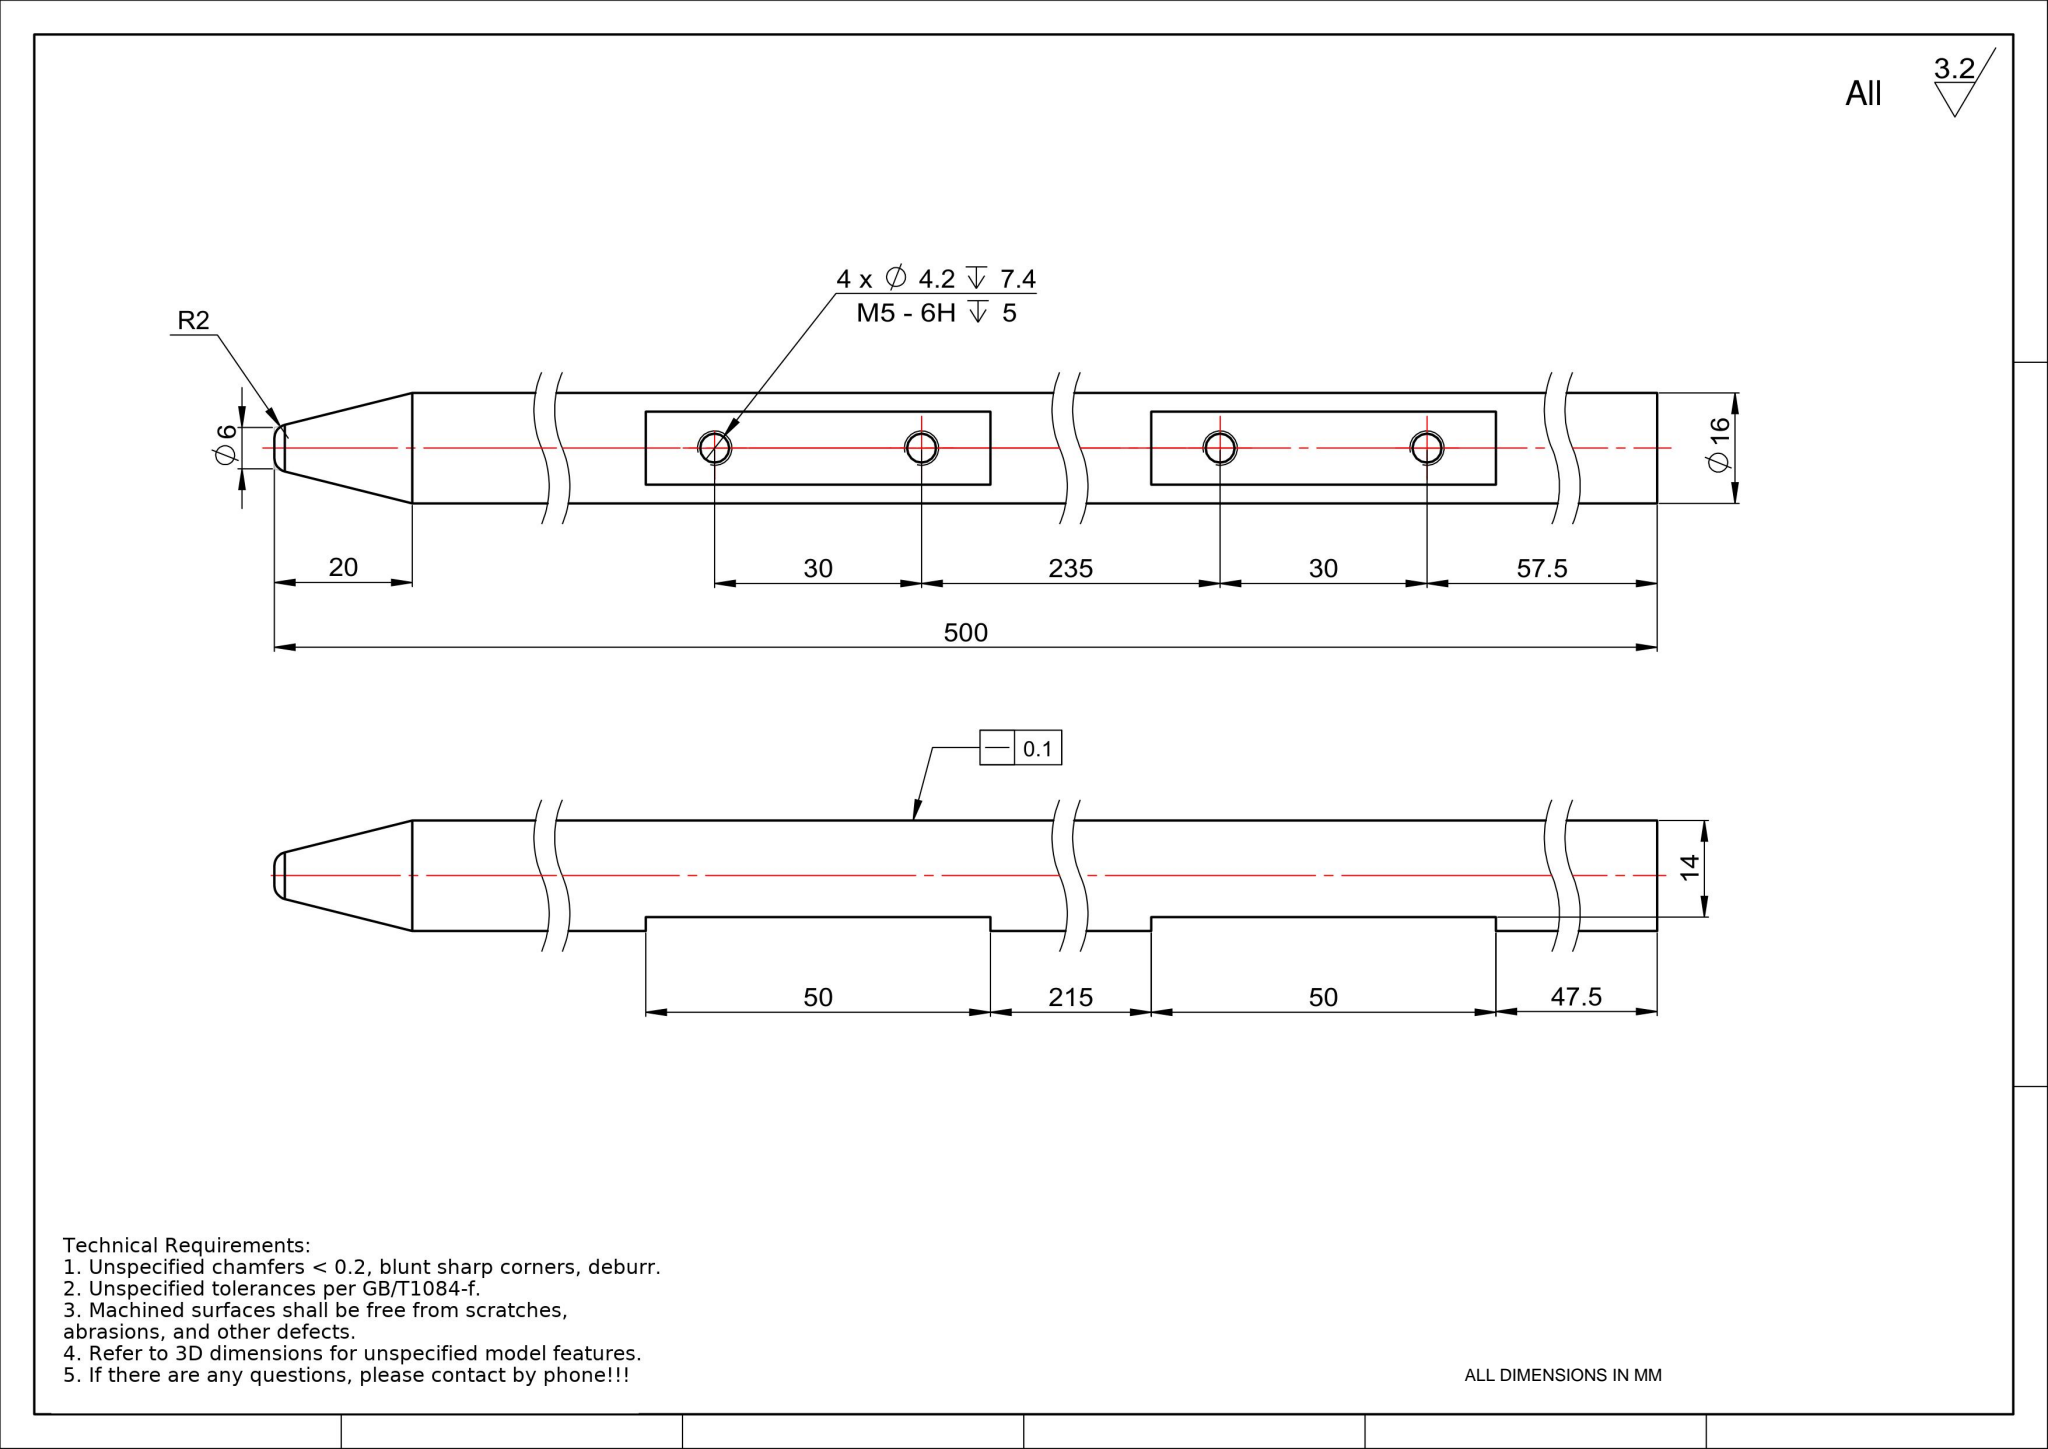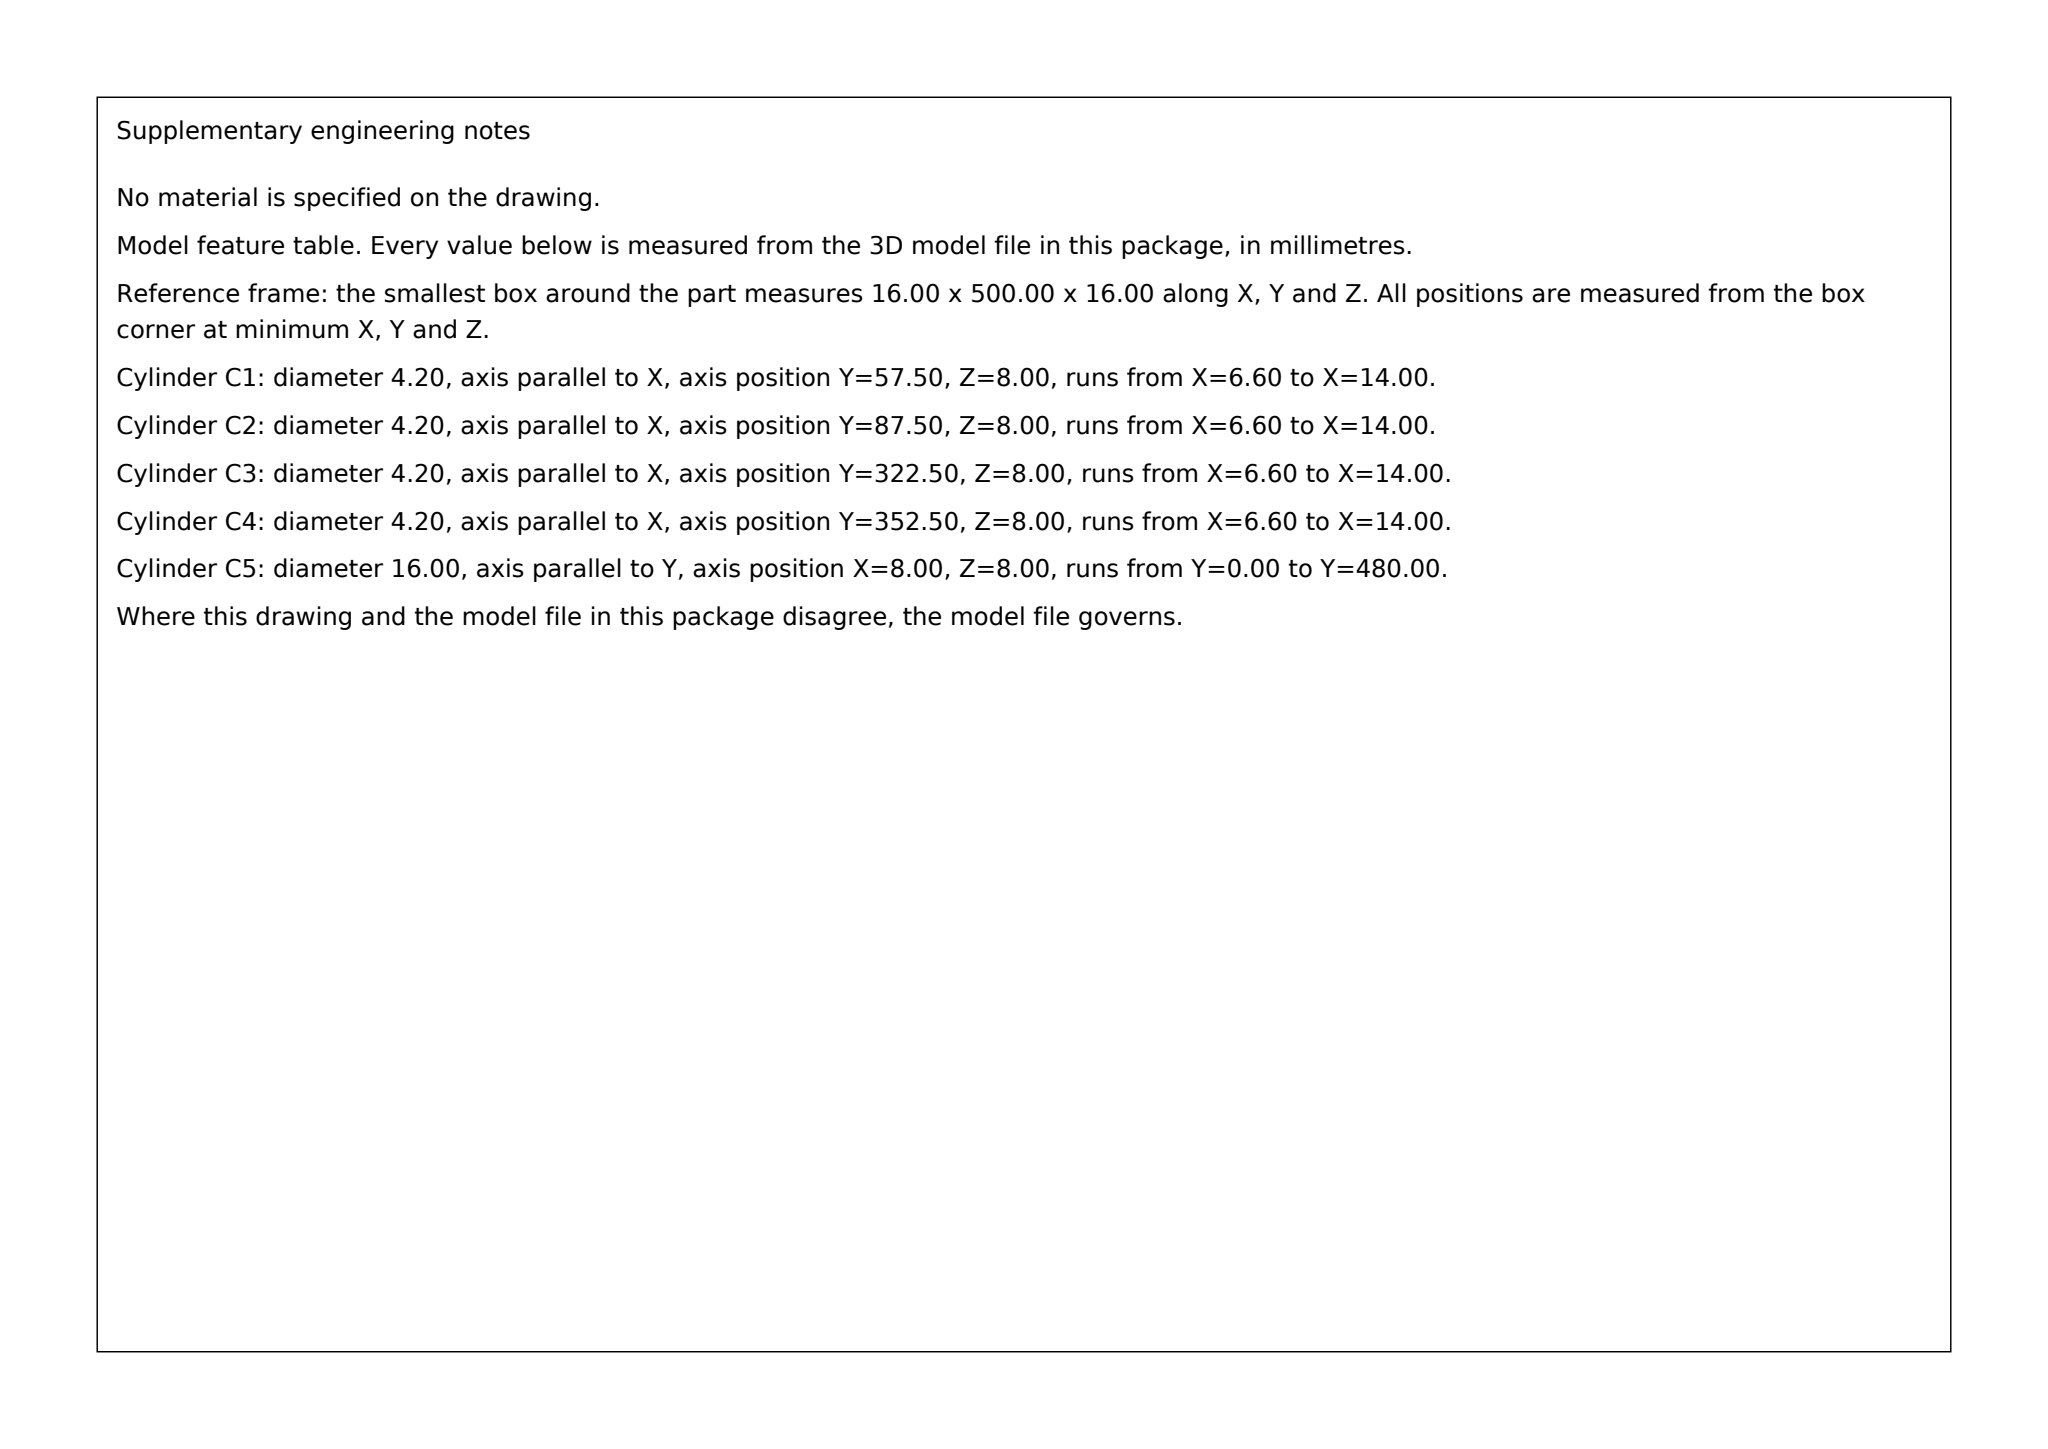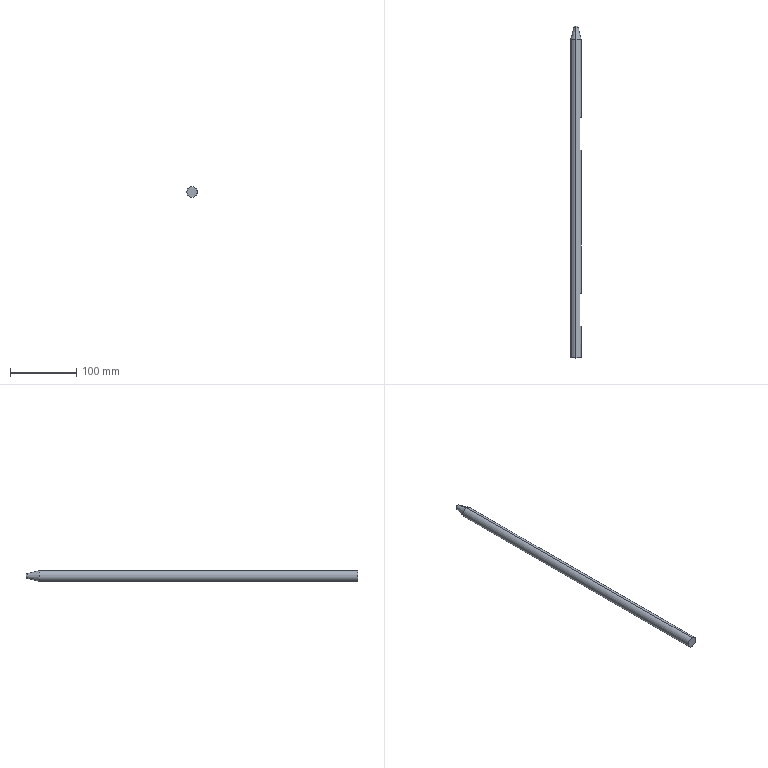Part | SolidWorks | mm | 1 solid | 30 faces | box 16 x 500 x 16 mm | volume 96649 mm3 | cylinder 10 | cone 10 | plane 8 | torus 2 | commonest cylinder face diameters 4.2 x8 16 x2
build123d program:
from build123d import *

# Parameters (mm, degrees)
SKETCH1_R                  = 8
BOSS_EXTRUDE1_DEPTH        = 500
CHAMFER2_SIZE              = 20
CHAMFER2_SIZE2             = 5
CUT_EXTRUDE1_START         = 6
SKETCH2_W                  = 36.807
SKETCH2_H                  = 50
CUT_EXTRUDE1_DEPTH         = 11
M5_TAPPED_HOLE1_AT_2_COUNT = 2
M5_TAPPED_HOLE1_AT_2_PITCH = 30
FILLET1_R                  = 2
LPATTERN3_COUNT            = 2
LPATTERN3_PITCH            = 265


with BuildPart() as part:
    # Sketch1 → Boss-Extrude1 (new body)
    with BuildSketch(Plane(origin=(0, 0, 0), x_dir=(1, 0, 0), z_dir=(0, 1, 0))):
        with Locations(Location((0, 0, 0), (0, 0, 270))):
            Circle(SKETCH1_R)
    extrude(amount=BOSS_EXTRUDE1_DEPTH)

    # Chamfer2
    chamfer2_edges = [part.edges().sort_by_distance(p)[0] for p in [
        (0, 500, -8),
    ]]
    chamfer2_side = [part.faces().sort_by_distance(p)[0] for p in [
        (0, 250, -8),
    ]]
    chamfer(chamfer2_edges, length=CHAMFER2_SIZE, length2=CHAMFER2_SIZE2, reference=chamfer2_side[0])

    # Sketch2 → Cut-Extrude1 (cut)
    with BuildSketch(Plane(origin=(0, 0, 0), x_dir=(0, 0, -1), z_dir=(1, 0, 0)).offset(CUT_EXTRUDE1_START)):
        with Locations((0, 72.5)):
            Rectangle(SKETCH2_W, SKETCH2_H)
    cut_extrude1 = extrude(amount=CUT_EXTRUDE1_DEPTH, mode=Mode.SUBTRACT)

    # Sketch3 → M5 Tapped Hole1 (revolve, cut)
    with BuildSketch(Plane(origin=(6, 87.5, 0), x_dir=(0, 0, -1), z_dir=(0, 1, 0))):
        Polygon((0, 0), (0, 8.662), (2.1, 7.4), (2.1, 0), align=None)
    m5_tapped_hole1 = revolve(axis=Axis((12.35, 87.5, 0), (-1, 0, 0)), mode=Mode.SUBTRACT)

    # M5 Tapped Hole1 at 2: M5 Tapped Hole1 ×2
    with Locations(*[(0, -i * M5_TAPPED_HOLE1_AT_2_PITCH, 0) for i in range(1, M5_TAPPED_HOLE1_AT_2_COUNT)]):
        add(m5_tapped_hole1, mode=Mode.SUBTRACT)

    # Fillet1
    fillet1_edges = [part.edges().sort_by_distance(p)[0] for p in [
        (0, 500, -3),
    ]]
    fillet(fillet1_edges, radius=FILLET1_R)

    # LPattern3: Cut-Extrude1, M5 Tapped Hole1 ×2
    with Locations(*[(0, i * LPATTERN3_PITCH, 0) for i in range(1, LPATTERN3_COUNT)]):
        add(cut_extrude1, mode=Mode.SUBTRACT)
        add(m5_tapped_hole1, mode=Mode.SUBTRACT)

    # LPattern3 copy 1 sketch → LPattern3 copy 1 (revolve, cut)
    with BuildSketch(Plane(origin=(6, 322.5, 0), x_dir=(0, 0, -1), z_dir=(0, 1, 0))):
        Polygon((0, 0), (0, 8.662), (2.1, 7.4), (2.1, 0), align=None)
    revolve(axis=Axis((12.35, 322.5, 0), (-1, 0, 0)), mode=Mode.SUBTRACT)


solid = part.part
STEP:
#1=CARTESIAN_POINT('',(-1.4,352.5,2.1));
#2=VERTEX_POINT('',#1);
#3=CARTESIAN_POINT('',(-1.4,352.5,-2.1));
#4=VERTEX_POINT('',#3);
#5=CARTESIAN_POINT('',(-1.4,352.5,0.));
#6=DIRECTION('',(1.,0.,0.));
#7=DIRECTION('',(0.,0.,-1.));
#8=AXIS2_PLACEMENT_3D('',#5,#6,#7);
#9=CIRCLE('',#8,2.1);
#10=EDGE_CURVE('',#2,#4,#9,.T.);
#11=ORIENTED_EDGE('',*,*,#10,.F.);
#12=CARTESIAN_POINT('',(6.,352.5,2.1));
#13=VERTEX_POINT('',#12);
#14=CARTESIAN_POINT('',(6.,352.5,2.1));
#15=DIRECTION('',(1.,0.,0.));
#16=VECTOR('',#15,1000.);
#17=LINE('',#14,#16);
#18=EDGE_CURVE('',#2,#13,#17,.T.);
#19=ORIENTED_EDGE('',*,*,#18,.T.);
#20=CARTESIAN_POINT('',(6.,352.5,-2.1));
#21=VERTEX_POINT('',#20);
#22=CARTESIAN_POINT('',(6.,352.5,0.));
#23=DIRECTION('',(1.,0.,0.));
#24=DIRECTION('',(0.,0.,-1.));
#25=AXIS2_PLACEMENT_3D('',#22,#23,#24);
#26=CIRCLE('',#25,2.1);
#27=EDGE_CURVE('',#13,#21,#26,.T.);
#28=ORIENTED_EDGE('',*,*,#27,.T.);
#29=CARTESIAN_POINT('',(6.,352.5,-2.1));
#30=DIRECTION('',(1.,0.,0.));
#31=VECTOR('',#30,1000.);
#32=LINE('',#29,#31);
#33=EDGE_CURVE('',#4,#21,#32,.T.);
#34=ORIENTED_EDGE('',*,*,#33,.F.);
#35=EDGE_LOOP('',(#11,#19,#28,#34));
#36=FACE_OUTER_BOUND('',#35,.T.);
#37=CARTESIAN_POINT('',(6.,352.5,0.));
#38=DIRECTION('',(1.,0.,0.));
#39=DIRECTION('',(0.,0.,-1.));
#40=AXIS2_PLACEMENT_3D('',#37,#38,#39);
#41=CYLINDRICAL_SURFACE('',#40,2.1);
#42=ADVANCED_FACE('',(#36),#41,.F.);
#43=CARTESIAN_POINT('',(-2.662,352.5,0.));
#44=VERTEX_POINT('',#43);
#45=CARTESIAN_POINT('',(-1.4,352.5,-2.1));
#46=DIRECTION('',(0.515,0.,-0.8572));
#47=VECTOR('',#46,1000.);
#48=LINE('',#45,#47);
#49=EDGE_CURVE('',#44,#4,#48,.T.);
#50=ORIENTED_EDGE('',*,*,#49,.F.);
#51=CARTESIAN_POINT('',(-1.4,352.5,2.1));
#52=DIRECTION('',(0.515,0.,0.8572));
#53=VECTOR('',#52,1000.);
#54=LINE('',#51,#53);
#55=EDGE_CURVE('',#44,#2,#54,.T.);
#56=ORIENTED_EDGE('',*,*,#55,.T.);
#57=ORIENTED_EDGE('',*,*,#10,.T.);
#58=EDGE_LOOP('',(#50,#56,#57));
#59=FACE_OUTER_BOUND('',#58,.T.);
#60=CARTESIAN_POINT('',(-1.4,352.5,0.));
#61=DIRECTION('',(1.,0.,0.));
#62=DIRECTION('',(0.,0.,-1.));
#63=AXIS2_PLACEMENT_3D('',#60,#61,#62);
#64=CONICAL_SURFACE('',#63,2.1,1.03);
#65=ADVANCED_FACE('',(#59),#64,.F.);
#66=CARTESIAN_POINT('',(-1.4,322.5,2.1));
#67=VERTEX_POINT('',#66);
#68=CARTESIAN_POINT('',(-1.4,322.5,-2.1));
#69=VERTEX_POINT('',#68);
#70=CARTESIAN_POINT('',(-1.4,322.5,0.));
#71=DIRECTION('',(1.,0.,0.));
#72=DIRECTION('',(0.,0.,-1.));
#73=AXIS2_PLACEMENT_3D('',#70,#71,#72);
#74=CIRCLE('',#73,2.1);
#75=EDGE_CURVE('',#67,#69,#74,.T.);
#76=ORIENTED_EDGE('',*,*,#75,.F.);
#77=CARTESIAN_POINT('',(6.,322.5,2.1));
#78=VERTEX_POINT('',#77);
#79=CARTESIAN_POINT('',(6.,322.5,2.1));
#80=DIRECTION('',(1.,0.,0.));
#81=VECTOR('',#80,1000.);
#82=LINE('',#79,#81);
#83=EDGE_CURVE('',#67,#78,#82,.T.);
#84=ORIENTED_EDGE('',*,*,#83,.T.);
#85=CARTESIAN_POINT('',(6.,322.5,-2.1));
#86=VERTEX_POINT('',#85);
#87=CARTESIAN_POINT('',(6.,322.5,0.));
#88=DIRECTION('',(1.,0.,0.));
#89=DIRECTION('',(0.,0.,-1.));
#90=AXIS2_PLACEMENT_3D('',#87,#88,#89);
#91=CIRCLE('',#90,2.1);
#92=EDGE_CURVE('',#78,#86,#91,.T.);
#93=ORIENTED_EDGE('',*,*,#92,.T.);
#94=CARTESIAN_POINT('',(6.,322.5,-2.1));
#95=DIRECTION('',(1.,0.,0.));
#96=VECTOR('',#95,1000.);
#97=LINE('',#94,#96);
#98=EDGE_CURVE('',#69,#86,#97,.T.);
#99=ORIENTED_EDGE('',*,*,#98,.F.);
#100=EDGE_LOOP('',(#76,#84,#93,#99));
#101=FACE_OUTER_BOUND('',#100,.T.);
#102=CARTESIAN_POINT('',(6.,322.5,0.));
#103=DIRECTION('',(1.,0.,0.));
#104=DIRECTION('',(0.,0.,-1.));
#105=AXIS2_PLACEMENT_3D('',#102,#103,#104);
#106=CYLINDRICAL_SURFACE('',#105,2.1);
#107=ADVANCED_FACE('',(#101),#106,.F.);
#108=CARTESIAN_POINT('',(-2.662,322.5,0.));
#109=VERTEX_POINT('',#108);
#110=CARTESIAN_POINT('',(-1.4,322.5,-2.1));
#111=DIRECTION('',(0.515,0.,-0.8572));
#112=VECTOR('',#111,1000.);
#113=LINE('',#110,#112);
#114=EDGE_CURVE('',#109,#69,#113,.T.);
#115=ORIENTED_EDGE('',*,*,#114,.F.);
#116=CARTESIAN_POINT('',(-1.4,322.5,2.1));
#117=DIRECTION('',(0.515,0.,0.8572));
#118=VECTOR('',#117,1000.);
#119=LINE('',#116,#118);
#120=EDGE_CURVE('',#109,#67,#119,.T.);
#121=ORIENTED_EDGE('',*,*,#120,.T.);
#122=ORIENTED_EDGE('',*,*,#75,.T.);
#123=EDGE_LOOP('',(#115,#121,#122));
#124=FACE_OUTER_BOUND('',#123,.T.);
#125=CARTESIAN_POINT('',(-1.4,322.5,0.));
#126=DIRECTION('',(1.,0.,0.));
#127=DIRECTION('',(0.,0.,-1.));
#128=AXIS2_PLACEMENT_3D('',#125,#126,#127);
#129=CONICAL_SURFACE('',#128,2.1,1.03);
#130=ADVANCED_FACE('',(#124),#129,.F.);
#131=CARTESIAN_POINT('',(0.,498.485,-3.379));
#132=VERTEX_POINT('',#131);
#133=CARTESIAN_POINT('',(0.,498.485,3.379));
#134=VERTEX_POINT('',#133);
#135=CARTESIAN_POINT('',(0.,498.485,0.));
#136=DIRECTION('',(0.,-1.,0.));
#137=DIRECTION('',(0.,0.,1.));
#138=AXIS2_PLACEMENT_3D('',#135,#136,#137);
#139=CIRCLE('',#138,3.379);
#140=EDGE_CURVE('',#132,#134,#139,.T.);
#141=ORIENTED_EDGE('',*,*,#140,.F.);
#142=CARTESIAN_POINT('',(0.,500.,-1.438));
#143=VERTEX_POINT('',#142);
#144=CARTESIAN_POINT('',(0.,498.,-1.438));
#145=DIRECTION('',(1.,0.,0.));
#146=DIRECTION('',(0.,0.,-1.));
#147=AXIS2_PLACEMENT_3D('',#144,#145,#146);
#148=CIRCLE('',#147,2.);
#149=EDGE_CURVE('',#132,#143,#148,.T.);
#150=ORIENTED_EDGE('',*,*,#149,.T.);
#151=CARTESIAN_POINT('',(0.,500.,1.438));
#152=VERTEX_POINT('',#151);
#153=CARTESIAN_POINT('',(0.,500.,0.));
#154=DIRECTION('',(0.,1.,0.));
#155=DIRECTION('',(0.,0.,1.));
#156=AXIS2_PLACEMENT_3D('',#153,#154,#155);
#157=CIRCLE('',#156,1.438);
#158=EDGE_CURVE('',#152,#143,#157,.T.);
#159=ORIENTED_EDGE('',*,*,#158,.F.);
#160=CARTESIAN_POINT('',(0.,498.,1.438));
#161=DIRECTION('',(-1.,0.,0.));
#162=DIRECTION('',(0.,0.,1.));
#163=AXIS2_PLACEMENT_3D('',#160,#161,#162);
#164=CIRCLE('',#163,2.);
#165=EDGE_CURVE('',#134,#152,#164,.T.);
#166=ORIENTED_EDGE('',*,*,#165,.F.);
#167=EDGE_LOOP('',(#141,#150,#159,#166));
#168=FACE_OUTER_BOUND('',#167,.T.);
#169=CARTESIAN_POINT('',(0.,498.,0.));
#170=DIRECTION('',(0.,1.,0.));
#171=DIRECTION('',(0.,0.,1.));
#172=AXIS2_PLACEMENT_3D('',#169,#170,#171);
#173=TOROIDAL_SURFACE('',#172,1.438,2.);
#174=ADVANCED_FACE('',(#168),#173,.T.);
#175=CARTESIAN_POINT('',(-1.4,87.5,2.1));
#176=VERTEX_POINT('',#175);
#177=CARTESIAN_POINT('',(-1.4,87.5,-2.1));
#178=VERTEX_POINT('',#177);
#179=CARTESIAN_POINT('',(-1.4,87.5,0.));
#180=DIRECTION('',(1.,0.,0.));
#181=DIRECTION('',(0.,0.,-1.));
#182=AXIS2_PLACEMENT_3D('',#179,#180,#181);
#183=CIRCLE('',#182,2.1);
#184=EDGE_CURVE('',#176,#178,#183,.T.);
#185=ORIENTED_EDGE('',*,*,#184,.F.);
#186=CARTESIAN_POINT('',(6.,87.5,2.1));
#187=VERTEX_POINT('',#186);
#188=CARTESIAN_POINT('',(6.,87.5,2.1));
#189=DIRECTION('',(1.,0.,0.));
#190=VECTOR('',#189,1000.);
#191=LINE('',#188,#190);
#192=EDGE_CURVE('',#176,#187,#191,.T.);
#193=ORIENTED_EDGE('',*,*,#192,.T.);
#194=CARTESIAN_POINT('',(6.,87.5,-2.1));
#195=VERTEX_POINT('',#194);
#196=CARTESIAN_POINT('',(6.,87.5,0.));
#197=DIRECTION('',(1.,0.,0.));
#198=DIRECTION('',(0.,0.,-1.));
#199=AXIS2_PLACEMENT_3D('',#196,#197,#198);
#200=CIRCLE('',#199,2.1);
#201=EDGE_CURVE('',#187,#195,#200,.T.);
#202=ORIENTED_EDGE('',*,*,#201,.T.);
#203=CARTESIAN_POINT('',(6.,87.5,-2.1));
#204=DIRECTION('',(1.,0.,0.));
#205=VECTOR('',#204,1000.);
#206=LINE('',#203,#205);
#207=EDGE_CURVE('',#178,#195,#206,.T.);
#208=ORIENTED_EDGE('',*,*,#207,.F.);
#209=EDGE_LOOP('',(#185,#193,#202,#208));
#210=FACE_OUTER_BOUND('',#209,.T.);
#211=CARTESIAN_POINT('',(6.,87.5,0.));
#212=DIRECTION('',(1.,0.,0.));
#213=DIRECTION('',(0.,0.,-1.));
#214=AXIS2_PLACEMENT_3D('',#211,#212,#213);
#215=CYLINDRICAL_SURFACE('',#214,2.1);
#216=ADVANCED_FACE('',(#210),#215,.F.);
#217=CARTESIAN_POINT('',(-2.662,87.5,0.));
#218=VERTEX_POINT('',#217);
#219=CARTESIAN_POINT('',(-1.4,87.5,-2.1));
#220=DIRECTION('',(0.515,0.,-0.8572));
#221=VECTOR('',#220,1000.);
#222=LINE('',#219,#221);
#223=EDGE_CURVE('',#218,#178,#222,.T.);
#224=ORIENTED_EDGE('',*,*,#223,.F.);
#225=CARTESIAN_POINT('',(-1.4,87.5,2.1));
#226=DIRECTION('',(0.515,0.,0.8572));
#227=VECTOR('',#226,1000.);
#228=LINE('',#225,#227);
#229=EDGE_CURVE('',#218,#176,#228,.T.);
#230=ORIENTED_EDGE('',*,*,#229,.T.);
#231=ORIENTED_EDGE('',*,*,#184,.T.);
#232=EDGE_LOOP('',(#224,#230,#231));
#233=FACE_OUTER_BOUND('',#232,.T.);
#234=CARTESIAN_POINT('',(-1.4,87.5,0.));
#235=DIRECTION('',(1.,0.,0.));
#236=DIRECTION('',(0.,0.,-1.));
#237=AXIS2_PLACEMENT_3D('',#234,#235,#236);
#238=CONICAL_SURFACE('',#237,2.1,1.03);
#239=ADVANCED_FACE('',(#233),#238,.F.);
#240=CARTESIAN_POINT('',(-1.4,57.5,2.1));
#241=VERTEX_POINT('',#240);
#242=CARTESIAN_POINT('',(-1.4,57.5,-2.1));
#243=VERTEX_POINT('',#242);
#244=CARTESIAN_POINT('',(-1.4,57.5,0.));
#245=DIRECTION('',(1.,0.,0.));
#246=DIRECTION('',(0.,0.,-1.));
#247=AXIS2_PLACEMENT_3D('',#244,#245,#246);
#248=CIRCLE('',#247,2.1);
#249=EDGE_CURVE('',#241,#243,#248,.T.);
#250=ORIENTED_EDGE('',*,*,#249,.F.);
#251=CARTESIAN_POINT('',(6.,57.5,2.1));
#252=VERTEX_POINT('',#251);
#253=CARTESIAN_POINT('',(6.,57.5,2.1));
#254=DIRECTION('',(1.,0.,0.));
#255=VECTOR('',#254,1000.);
#256=LINE('',#253,#255);
#257=EDGE_CURVE('',#241,#252,#256,.T.);
#258=ORIENTED_EDGE('',*,*,#257,.T.);
#259=CARTESIAN_POINT('',(6.,57.5,-2.1));
#260=VERTEX_POINT('',#259);
#261=CARTESIAN_POINT('',(6.,57.5,0.));
#262=DIRECTION('',(1.,0.,0.));
#263=DIRECTION('',(0.,0.,-1.));
#264=AXIS2_PLACEMENT_3D('',#261,#262,#263);
#265=CIRCLE('',#264,2.1);
#266=EDGE_CURVE('',#252,#260,#265,.T.);
#267=ORIENTED_EDGE('',*,*,#266,.T.);
#268=CARTESIAN_POINT('',(6.,57.5,-2.1));
#269=DIRECTION('',(1.,0.,0.));
#270=VECTOR('',#269,1000.);
#271=LINE('',#268,#270);
#272=EDGE_CURVE('',#243,#260,#271,.T.);
#273=ORIENTED_EDGE('',*,*,#272,.F.);
#274=EDGE_LOOP('',(#250,#258,#267,#273));
#275=FACE_OUTER_BOUND('',#274,.T.);
#276=CARTESIAN_POINT('',(6.,57.5,0.));
#277=DIRECTION('',(1.,0.,0.));
#278=DIRECTION('',(0.,0.,-1.));
#279=AXIS2_PLACEMENT_3D('',#276,#277,#278);
#280=CYLINDRICAL_SURFACE('',#279,2.1);
#281=ADVANCED_FACE('',(#275),#280,.F.);
#282=CARTESIAN_POINT('',(-2.662,57.5,0.));
#283=VERTEX_POINT('',#282);
#284=CARTESIAN_POINT('',(-1.4,57.5,-2.1));
#285=DIRECTION('',(0.515,0.,-0.8572));
#286=VECTOR('',#285,1000.);
#287=LINE('',#284,#286);
#288=EDGE_CURVE('',#283,#243,#287,.T.);
#289=ORIENTED_EDGE('',*,*,#288,.F.);
#290=CARTESIAN_POINT('',(-1.4,57.5,2.1));
#291=DIRECTION('',(0.515,0.,0.8572));
#292=VECTOR('',#291,1000.);
#293=LINE('',#290,#292);
#294=EDGE_CURVE('',#283,#241,#293,.T.);
#295=ORIENTED_EDGE('',*,*,#294,.T.);
#296=ORIENTED_EDGE('',*,*,#249,.T.);
#297=EDGE_LOOP('',(#289,#295,#296));
#298=FACE_OUTER_BOUND('',#297,.T.);
#299=CARTESIAN_POINT('',(-1.4,57.5,0.));
#300=DIRECTION('',(1.,0.,0.));
#301=DIRECTION('',(0.,0.,-1.));
#302=AXIS2_PLACEMENT_3D('',#299,#300,#301);
#303=CONICAL_SURFACE('',#302,2.1,1.03);
#304=ADVANCED_FACE('',(#298),#303,.F.);
#305=ORIENTED_EDGE('',*,*,#140,.T.);
#306=CARTESIAN_POINT('',(0.,480.,8.));
#307=VERTEX_POINT('',#306);
#308=CARTESIAN_POINT('',(0.,500.,3.));
#309=DIRECTION('',(0.,-0.9701,0.2425));
#310=VECTOR('',#309,1000.);
#311=LINE('',#308,#310);
#312=EDGE_CURVE('',#134,#307,#311,.T.);
#313=ORIENTED_EDGE('',*,*,#312,.T.);
#314=CARTESIAN_POINT('',(0.,480.,-8.));
#315=VERTEX_POINT('',#314);
#316=CARTESIAN_POINT('',(0.,480.,0.));
#317=DIRECTION('',(0.,-1.,0.));
#318=DIRECTION('',(0.,0.,1.));
#319=AXIS2_PLACEMENT_3D('',#316,#317,#318);
#320=CIRCLE('',#319,8.);
#321=EDGE_CURVE('',#315,#307,#320,.T.);
#322=ORIENTED_EDGE('',*,*,#321,.F.);
#323=CARTESIAN_POINT('',(0.,500.,-3.));
#324=DIRECTION('',(0.,-0.9701,-0.2425));
#325=VECTOR('',#324,1000.);
#326=LINE('',#323,#325);
#327=EDGE_CURVE('',#132,#315,#326,.T.);
#328=ORIENTED_EDGE('',*,*,#327,.F.);
#329=EDGE_LOOP('',(#305,#313,#322,#328));
#330=FACE_OUTER_BOUND('',#329,.T.);
#331=CARTESIAN_POINT('',(0.,500.,0.));
#332=DIRECTION('',(0.,-1.,0.));
#333=DIRECTION('',(0.,0.,-1.));
#334=AXIS2_PLACEMENT_3D('',#331,#332,#333);
#335=CONICAL_SURFACE('',#334,3.,0.245);
#336=ADVANCED_FACE('',(#330),#335,.T.);
#337=CARTESIAN_POINT('',(6.,97.5,5.292));
#338=VERTEX_POINT('',#337);
#339=CARTESIAN_POINT('',(6.,47.5,5.292));
#340=VERTEX_POINT('',#339);
#341=CARTESIAN_POINT('',(6.,500.,5.292));
#342=DIRECTION('',(0.,-1.,0.));
#343=VECTOR('',#342,1000.);
#344=LINE('',#341,#343);
#345=EDGE_CURVE('',#338,#340,#344,.T.);
#346=ORIENTED_EDGE('',*,*,#345,.F.);
#347=CARTESIAN_POINT('',(6.,97.5,-5.292));
#348=VERTEX_POINT('',#347);
#349=CARTESIAN_POINT('',(0.,97.5,0.));
#350=DIRECTION('',(0.,-1.,0.));
#351=DIRECTION('',(0.,0.,-1.));
#352=AXIS2_PLACEMENT_3D('',#349,#350,#351);
#353=CIRCLE('',#352,8.);
#354=EDGE_CURVE('',#348,#338,#353,.T.);
#355=ORIENTED_EDGE('',*,*,#354,.F.);
#356=CARTESIAN_POINT('',(6.,47.5,-5.292));
#357=VERTEX_POINT('',#356);
#358=CARTESIAN_POINT('',(6.,500.,-5.292));
#359=DIRECTION('',(0.,1.,0.));
#360=VECTOR('',#359,1000.);
#361=LINE('',#358,#360);
#362=EDGE_CURVE('',#357,#348,#361,.T.);
#363=ORIENTED_EDGE('',*,*,#362,.F.);
#364=CARTESIAN_POINT('',(0.,47.5,0.));
#365=DIRECTION('',(0.,1.,0.));
#366=DIRECTION('',(0.,0.,1.));
#367=AXIS2_PLACEMENT_3D('',#364,#365,#366);
#368=CIRCLE('',#367,8.);
#369=EDGE_CURVE('',#340,#357,#368,.T.);
#370=ORIENTED_EDGE('',*,*,#369,.F.);
#371=EDGE_LOOP('',(#346,#355,#363,#370));
#372=FACE_BOUND('',#371,.T.);
#373=CARTESIAN_POINT('',(6.,362.5,5.292));
#374=VERTEX_POINT('',#373);
#375=CARTESIAN_POINT('',(6.,312.5,5.292));
#376=VERTEX_POINT('',#375);
#377=CARTESIAN_POINT('',(6.,500.,5.292));
#378=DIRECTION('',(0.,-1.,0.));
#379=VECTOR('',#378,1000.);
#380=LINE('',#377,#379);
#381=EDGE_CURVE('',#374,#376,#380,.T.);
#382=ORIENTED_EDGE('',*,*,#381,.F.);
#383=CARTESIAN_POINT('',(6.,362.5,-5.292));
#384=VERTEX_POINT('',#383);
#385=CARTESIAN_POINT('',(0.,362.5,0.));
#386=DIRECTION('',(0.,-1.,0.));
#387=DIRECTION('',(0.,0.,-1.));
#388=AXIS2_PLACEMENT_3D('',#385,#386,#387);
#389=CIRCLE('',#388,8.);
#390=EDGE_CURVE('',#384,#374,#389,.T.);
#391=ORIENTED_EDGE('',*,*,#390,.F.);
#392=CARTESIAN_POINT('',(6.,312.5,-5.292));
#393=VERTEX_POINT('',#392);
#394=CARTESIAN_POINT('',(6.,500.,-5.292));
#395=DIRECTION('',(0.,1.,0.));
#396=VECTOR('',#395,1000.);
#397=LINE('',#394,#396);
#398=EDGE_CURVE('',#393,#384,#397,.T.);
#399=ORIENTED_EDGE('',*,*,#398,.F.);
#400=CARTESIAN_POINT('',(0.,312.5,0.));
#401=DIRECTION('',(0.,1.,0.));
#402=DIRECTION('',(0.,0.,1.));
#403=AXIS2_PLACEMENT_3D('',#400,#401,#402);
#404=CIRCLE('',#403,8.);
#405=EDGE_CURVE('',#376,#393,#404,.T.);
#406=ORIENTED_EDGE('',*,*,#405,.F.);
#407=EDGE_LOOP('',(#382,#391,#399,#406));
#408=FACE_BOUND('',#407,.T.);
#409=ORIENTED_EDGE('',*,*,#321,.T.);
#410=CARTESIAN_POINT('',(0.,0.,8.));
#411=VERTEX_POINT('',#410);
#412=CARTESIAN_POINT('',(0.,500.,8.));
#413=DIRECTION('',(0.,-1.,0.));
#414=VECTOR('',#413,1000.);
#415=LINE('',#412,#414);
#416=EDGE_CURVE('',#307,#411,#415,.T.);
#417=ORIENTED_EDGE('',*,*,#416,.T.);
#418=CARTESIAN_POINT('',(0.,0.,-8.));
#419=VERTEX_POINT('',#418);
#420=CARTESIAN_POINT('',(0.,0.,0.));
#421=DIRECTION('',(0.,1.,0.));
#422=DIRECTION('',(0.,0.,1.));
#423=AXIS2_PLACEMENT_3D('',#420,#421,#422);
#424=CIRCLE('',#423,8.);
#425=EDGE_CURVE('',#411,#419,#424,.T.);
#426=ORIENTED_EDGE('',*,*,#425,.T.);
#427=CARTESIAN_POINT('',(0.,500.,-8.));
#428=DIRECTION('',(0.,-1.,0.));
#429=VECTOR('',#428,1000.);
#430=LINE('',#427,#429);
#431=EDGE_CURVE('',#315,#419,#430,.T.);
#432=ORIENTED_EDGE('',*,*,#431,.F.);
#433=EDGE_LOOP('',(#409,#417,#426,#432));
#434=FACE_OUTER_BOUND('',#433,.T.);
#435=CARTESIAN_POINT('',(0.,500.,0.));
#436=DIRECTION('',(0.,-1.,0.));
#437=DIRECTION('',(0.,0.,-1.));
#438=AXIS2_PLACEMENT_3D('',#435,#436,#437);
#439=CYLINDRICAL_SURFACE('',#438,8.);
#440=ADVANCED_FACE('',(#372,#408,#434),#439,.T.);
#441=ORIENTED_EDGE('',*,*,#416,.F.);
#442=CARTESIAN_POINT('',(0.,480.,0.));
#443=DIRECTION('',(0.,-1.,0.));
#444=DIRECTION('',(0.,0.,1.));
#445=AXIS2_PLACEMENT_3D('',#442,#443,#444);
#446=CIRCLE('',#445,8.);
#447=EDGE_CURVE('',#307,#315,#446,.T.);
#448=ORIENTED_EDGE('',*,*,#447,.T.);
#449=ORIENTED_EDGE('',*,*,#431,.T.);
#450=CARTESIAN_POINT('',(0.,0.,0.));
#451=DIRECTION('',(0.,1.,0.));
#452=DIRECTION('',(0.,0.,1.));
#453=AXIS2_PLACEMENT_3D('',#450,#451,#452);
#454=CIRCLE('',#453,8.);
#455=EDGE_CURVE('',#419,#411,#454,.T.);
#456=ORIENTED_EDGE('',*,*,#455,.T.);
#457=EDGE_LOOP('',(#441,#448,#449,#456));
#458=FACE_OUTER_BOUND('',#457,.T.);
#459=CARTESIAN_POINT('',(0.,500.,0.));
#460=DIRECTION('',(0.,-1.,0.));
#461=DIRECTION('',(0.,0.,-1.));
#462=AXIS2_PLACEMENT_3D('',#459,#460,#461);
#463=CYLINDRICAL_SURFACE('',#462,8.);
#464=ADVANCED_FACE('',(#458),#463,.T.);
#465=ORIENTED_EDGE('',*,*,#158,.T.);
#466=CARTESIAN_POINT('',(0.,500.,0.));
#467=DIRECTION('',(0.,1.,0.));
#468=DIRECTION('',(0.,0.,1.));
#469=AXIS2_PLACEMENT_3D('',#466,#467,#468);
#470=CIRCLE('',#469,1.438);
#471=EDGE_CURVE('',#143,#152,#470,.T.);
#472=ORIENTED_EDGE('',*,*,#471,.T.);
#473=EDGE_LOOP('',(#465,#472));
#474=FACE_OUTER_BOUND('',#473,.T.);
#475=CARTESIAN_POINT('',(0.,500.,0.));
#476=DIRECTION('',(0.,1.,0.));
#477=DIRECTION('',(0.,0.,1.));
#478=AXIS2_PLACEMENT_3D('',#475,#476,#477);
#479=PLANE('',#478);
#480=ADVANCED_FACE('',(#474),#479,.T.);
#481=ORIENTED_EDGE('',*,*,#455,.F.);
#482=ORIENTED_EDGE('',*,*,#425,.F.);
#483=EDGE_LOOP('',(#481,#482));
#484=FACE_OUTER_BOUND('',#483,.T.);
#485=CARTESIAN_POINT('',(0.,0.,0.));
#486=DIRECTION('',(0.,1.,0.));
#487=DIRECTION('',(0.,0.,1.));
#488=AXIS2_PLACEMENT_3D('',#485,#486,#487);
#489=PLANE('',#488);
#490=ADVANCED_FACE('',(#484),#489,.F.);
#491=ORIENTED_EDGE('',*,*,#312,.F.);
#492=CARTESIAN_POINT('',(0.,498.485,0.));
#493=DIRECTION('',(0.,-1.,0.));
#494=DIRECTION('',(0.,0.,1.));
#495=AXIS2_PLACEMENT_3D('',#492,#493,#494);
#496=CIRCLE('',#495,3.379);
#497=EDGE_CURVE('',#134,#132,#496,.T.);
#498=ORIENTED_EDGE('',*,*,#497,.T.);
#499=ORIENTED_EDGE('',*,*,#327,.T.);
#500=ORIENTED_EDGE('',*,*,#447,.F.);
#501=EDGE_LOOP('',(#491,#498,#499,#500));
#502=FACE_OUTER_BOUND('',#501,.T.);
#503=CARTESIAN_POINT('',(0.,500.,0.));
#504=DIRECTION('',(0.,-1.,0.));
#505=DIRECTION('',(0.,0.,-1.));
#506=AXIS2_PLACEMENT_3D('',#503,#504,#505);
#507=CONICAL_SURFACE('',#506,3.,0.245);
#508=ADVANCED_FACE('',(#502),#507,.T.);
#509=ORIENTED_EDGE('',*,*,#354,.T.);
#510=CARTESIAN_POINT('',(6.,97.5,18.403));
#511=DIRECTION('',(0.,0.,1.));
#512=VECTOR('',#511,1000.);
#513=LINE('',#510,#512);
#514=EDGE_CURVE('',#348,#338,#513,.T.);
#515=ORIENTED_EDGE('',*,*,#514,.F.);
#516=EDGE_LOOP('',(#509,#515));
#517=FACE_OUTER_BOUND('',#516,.T.);
#518=CARTESIAN_POINT('',(17.,97.5,18.403));
#519=DIRECTION('',(0.,-1.,0.));
#520=DIRECTION('',(0.,0.,-1.));
#521=AXIS2_PLACEMENT_3D('',#518,#519,#520);
#522=PLANE('',#521);
#523=ADVANCED_FACE('',(#517),#522,.T.);
#524=ORIENTED_EDGE('',*,*,#369,.T.);
#525=CARTESIAN_POINT('',(6.,47.5,18.403));
#526=DIRECTION('',(0.,0.,-1.));
#527=VECTOR('',#526,1000.);
#528=LINE('',#525,#527);
#529=EDGE_CURVE('',#340,#357,#528,.T.);
#530=ORIENTED_EDGE('',*,*,#529,.F.);
#531=EDGE_LOOP('',(#524,#530));
#532=FACE_OUTER_BOUND('',#531,.T.);
#533=CARTESIAN_POINT('',(17.,47.5,18.403));
#534=DIRECTION('',(0.,1.,0.));
#535=DIRECTION('',(0.,-0.,1.));
#536=AXIS2_PLACEMENT_3D('',#533,#534,#535);
#537=PLANE('',#536);
#538=ADVANCED_FACE('',(#532),#537,.T.);
#539=CARTESIAN_POINT('',(6.,87.5,0.));
#540=DIRECTION('',(1.,0.,0.));
#541=DIRECTION('',(0.,0.,-1.));
#542=AXIS2_PLACEMENT_3D('',#539,#540,#541);
#543=CIRCLE('',#542,2.1);
#544=EDGE_CURVE('',#195,#187,#543,.T.);
#545=ORIENTED_EDGE('',*,*,#544,.F.);
#546=ORIENTED_EDGE('',*,*,#201,.F.);
#547=EDGE_LOOP('',(#545,#546));
#548=FACE_BOUND('',#547,.T.);
#549=CARTESIAN_POINT('',(6.,57.5,0.));
#550=DIRECTION('',(1.,0.,0.));
#551=DIRECTION('',(0.,0.,-1.));
#552=AXIS2_PLACEMENT_3D('',#549,#550,#551);
#553=CIRCLE('',#552,2.1);
#554=EDGE_CURVE('',#260,#252,#553,.T.);
#555=ORIENTED_EDGE('',*,*,#554,.F.);
#556=ORIENTED_EDGE('',*,*,#266,.F.);
#557=EDGE_LOOP('',(#555,#556));
#558=FACE_BOUND('',#557,.T.);
#559=ORIENTED_EDGE('',*,*,#345,.T.);
#560=ORIENTED_EDGE('',*,*,#529,.T.);
#561=ORIENTED_EDGE('',*,*,#362,.T.);
#562=ORIENTED_EDGE('',*,*,#514,.T.);
#563=EDGE_LOOP('',(#559,#560,#561,#562));
#564=FACE_OUTER_BOUND('',#563,.T.);
#565=CARTESIAN_POINT('',(6.,0.,0.));
#566=DIRECTION('',(1.,0.,0.));
#567=DIRECTION('',(0.,0.,-1.));
#568=AXIS2_PLACEMENT_3D('',#565,#566,#567);
#569=PLANE('',#568);
#570=ADVANCED_FACE('',(#548,#558,#564),#569,.T.);
#571=ORIENTED_EDGE('',*,*,#294,.F.);
#572=ORIENTED_EDGE('',*,*,#288,.T.);
#573=CARTESIAN_POINT('',(-1.4,57.5,0.));
#574=DIRECTION('',(1.,0.,0.));
#575=DIRECTION('',(0.,0.,-1.));
#576=AXIS2_PLACEMENT_3D('',#573,#574,#575);
#577=CIRCLE('',#576,2.1);
#578=EDGE_CURVE('',#243,#241,#577,.T.);
#579=ORIENTED_EDGE('',*,*,#578,.T.);
#580=EDGE_LOOP('',(#571,#572,#579));
#581=FACE_OUTER_BOUND('',#580,.T.);
#582=CARTESIAN_POINT('',(-1.4,57.5,0.));
#583=DIRECTION('',(1.,0.,0.));
#584=DIRECTION('',(0.,0.,-1.));
#585=AXIS2_PLACEMENT_3D('',#582,#583,#584);
#586=CONICAL_SURFACE('',#585,2.1,1.03);
#587=ADVANCED_FACE('',(#581),#586,.F.);
#588=ORIENTED_EDGE('',*,*,#257,.F.);
#589=ORIENTED_EDGE('',*,*,#578,.F.);
#590=ORIENTED_EDGE('',*,*,#272,.T.);
#591=ORIENTED_EDGE('',*,*,#554,.T.);
#592=EDGE_LOOP('',(#588,#589,#590,#591));
#593=FACE_OUTER_BOUND('',#592,.T.);
#594=CARTESIAN_POINT('',(6.,57.5,0.));
#595=DIRECTION('',(1.,0.,0.));
#596=DIRECTION('',(0.,0.,-1.));
#597=AXIS2_PLACEMENT_3D('',#594,#595,#596);
#598=CYLINDRICAL_SURFACE('',#597,2.1);
#599=ADVANCED_FACE('',(#593),#598,.F.);
#600=ORIENTED_EDGE('',*,*,#229,.F.);
#601=ORIENTED_EDGE('',*,*,#223,.T.);
#602=CARTESIAN_POINT('',(-1.4,87.5,0.));
#603=DIRECTION('',(1.,0.,0.));
#604=DIRECTION('',(0.,0.,-1.));
#605=AXIS2_PLACEMENT_3D('',#602,#603,#604);
#606=CIRCLE('',#605,2.1);
#607=EDGE_CURVE('',#178,#176,#606,.T.);
#608=ORIENTED_EDGE('',*,*,#607,.T.);
#609=EDGE_LOOP('',(#600,#601,#608));
#610=FACE_OUTER_BOUND('',#609,.T.);
#611=CARTESIAN_POINT('',(-1.4,87.5,0.));
#612=DIRECTION('',(1.,0.,0.));
#613=DIRECTION('',(0.,0.,-1.));
#614=AXIS2_PLACEMENT_3D('',#611,#612,#613);
#615=CONICAL_SURFACE('',#614,2.1,1.03);
#616=ADVANCED_FACE('',(#610),#615,.F.);
#617=ORIENTED_EDGE('',*,*,#192,.F.);
#618=ORIENTED_EDGE('',*,*,#607,.F.);
#619=ORIENTED_EDGE('',*,*,#207,.T.);
#620=ORIENTED_EDGE('',*,*,#544,.T.);
#621=EDGE_LOOP('',(#617,#618,#619,#620));
#622=FACE_OUTER_BOUND('',#621,.T.);
#623=CARTESIAN_POINT('',(6.,87.5,0.));
#624=DIRECTION('',(1.,0.,0.));
#625=DIRECTION('',(0.,0.,-1.));
#626=AXIS2_PLACEMENT_3D('',#623,#624,#625);
#627=CYLINDRICAL_SURFACE('',#626,2.1);
#628=ADVANCED_FACE('',(#622),#627,.F.);
#629=ORIENTED_EDGE('',*,*,#149,.F.);
#630=ORIENTED_EDGE('',*,*,#497,.F.);
#631=ORIENTED_EDGE('',*,*,#165,.T.);
#632=ORIENTED_EDGE('',*,*,#471,.F.);
#633=EDGE_LOOP('',(#629,#630,#631,#632));
#634=FACE_OUTER_BOUND('',#633,.T.);
#635=CARTESIAN_POINT('',(0.,498.,0.));
#636=DIRECTION('',(0.,1.,0.));
#637=DIRECTION('',(0.,0.,1.));
#638=AXIS2_PLACEMENT_3D('',#635,#636,#637);
#639=TOROIDAL_SURFACE('',#638,1.438,2.);
#640=ADVANCED_FACE('',(#634),#639,.T.);
#641=ORIENTED_EDGE('',*,*,#390,.T.);
#642=CARTESIAN_POINT('',(6.,362.5,18.403));
#643=DIRECTION('',(0.,0.,1.));
#644=VECTOR('',#643,1000.);
#645=LINE('',#642,#644);
#646=EDGE_CURVE('',#384,#374,#645,.T.);
#647=ORIENTED_EDGE('',*,*,#646,.F.);
#648=EDGE_LOOP('',(#641,#647));
#649=FACE_OUTER_BOUND('',#648,.T.);
#650=CARTESIAN_POINT('',(17.,362.5,18.403));
#651=DIRECTION('',(0.,-1.,0.));
#652=DIRECTION('',(0.,0.,-1.));
#653=AXIS2_PLACEMENT_3D('',#650,#651,#652);
#654=PLANE('',#653);
#655=ADVANCED_FACE('',(#649),#654,.T.);
#656=ORIENTED_EDGE('',*,*,#405,.T.);
#657=CARTESIAN_POINT('',(6.,312.5,18.403));
#658=DIRECTION('',(0.,0.,-1.));
#659=VECTOR('',#658,1000.);
#660=LINE('',#657,#659);
#661=EDGE_CURVE('',#376,#393,#660,.T.);
#662=ORIENTED_EDGE('',*,*,#661,.F.);
#663=EDGE_LOOP('',(#656,#662));
#664=FACE_OUTER_BOUND('',#663,.T.);
#665=CARTESIAN_POINT('',(17.,312.5,18.403));
#666=DIRECTION('',(0.,1.,0.));
#667=DIRECTION('',(0.,-0.,1.));
#668=AXIS2_PLACEMENT_3D('',#665,#666,#667);
#669=PLANE('',#668);
#670=ADVANCED_FACE('',(#664),#669,.T.);
#671=CARTESIAN_POINT('',(6.,352.5,0.));
#672=DIRECTION('',(1.,0.,0.));
#673=DIRECTION('',(0.,0.,-1.));
#674=AXIS2_PLACEMENT_3D('',#671,#672,#673);
#675=CIRCLE('',#674,2.1);
#676=EDGE_CURVE('',#21,#13,#675,.T.);
#677=ORIENTED_EDGE('',*,*,#676,.F.);
#678=ORIENTED_EDGE('',*,*,#27,.F.);
#679=EDGE_LOOP('',(#677,#678));
#680=FACE_BOUND('',#679,.T.);
#681=CARTESIAN_POINT('',(6.,322.5,0.));
#682=DIRECTION('',(1.,0.,0.));
#683=DIRECTION('',(0.,0.,-1.));
#684=AXIS2_PLACEMENT_3D('',#681,#682,#683);
#685=CIRCLE('',#684,2.1);
#686=EDGE_CURVE('',#86,#78,#685,.T.);
#687=ORIENTED_EDGE('',*,*,#686,.F.);
#688=ORIENTED_EDGE('',*,*,#92,.F.);
#689=EDGE_LOOP('',(#687,#688));
#690=FACE_BOUND('',#689,.T.);
#691=ORIENTED_EDGE('',*,*,#381,.T.);
#692=ORIENTED_EDGE('',*,*,#661,.T.);
#693=ORIENTED_EDGE('',*,*,#398,.T.);
#694=ORIENTED_EDGE('',*,*,#646,.T.);
#695=EDGE_LOOP('',(#691,#692,#693,#694));
#696=FACE_OUTER_BOUND('',#695,.T.);
#697=CARTESIAN_POINT('',(6.,265.,0.));
#698=DIRECTION('',(1.,0.,0.));
#699=DIRECTION('',(0.,0.,-1.));
#700=AXIS2_PLACEMENT_3D('',#697,#698,#699);
#701=PLANE('',#700);
#702=ADVANCED_FACE('',(#680,#690,#696),#701,.T.);
#703=ORIENTED_EDGE('',*,*,#120,.F.);
#704=ORIENTED_EDGE('',*,*,#114,.T.);
#705=CARTESIAN_POINT('',(-1.4,322.5,0.));
#706=DIRECTION('',(1.,0.,0.));
#707=DIRECTION('',(0.,0.,-1.));
#708=AXIS2_PLACEMENT_3D('',#705,#706,#707);
#709=CIRCLE('',#708,2.1);
#710=EDGE_CURVE('',#69,#67,#709,.T.);
#711=ORIENTED_EDGE('',*,*,#710,.T.);
#712=EDGE_LOOP('',(#703,#704,#711));
#713=FACE_OUTER_BOUND('',#712,.T.);
#714=CARTESIAN_POINT('',(-1.4,322.5,0.));
#715=DIRECTION('',(1.,0.,0.));
#716=DIRECTION('',(0.,0.,-1.));
#717=AXIS2_PLACEMENT_3D('',#714,#715,#716);
#718=CONICAL_SURFACE('',#717,2.1,1.03);
#719=ADVANCED_FACE('',(#713),#718,.F.);
#720=ORIENTED_EDGE('',*,*,#83,.F.);
#721=ORIENTED_EDGE('',*,*,#710,.F.);
#722=ORIENTED_EDGE('',*,*,#98,.T.);
#723=ORIENTED_EDGE('',*,*,#686,.T.);
#724=EDGE_LOOP('',(#720,#721,#722,#723));
#725=FACE_OUTER_BOUND('',#724,.T.);
#726=CARTESIAN_POINT('',(6.,322.5,0.));
#727=DIRECTION('',(1.,0.,0.));
#728=DIRECTION('',(0.,0.,-1.));
#729=AXIS2_PLACEMENT_3D('',#726,#727,#728);
#730=CYLINDRICAL_SURFACE('',#729,2.1);
#731=ADVANCED_FACE('',(#725),#730,.F.);
#732=ORIENTED_EDGE('',*,*,#55,.F.);
#733=ORIENTED_EDGE('',*,*,#49,.T.);
#734=CARTESIAN_POINT('',(-1.4,352.5,0.));
#735=DIRECTION('',(1.,0.,0.));
#736=DIRECTION('',(0.,0.,-1.));
#737=AXIS2_PLACEMENT_3D('',#734,#735,#736);
#738=CIRCLE('',#737,2.1);
#739=EDGE_CURVE('',#4,#2,#738,.T.);
#740=ORIENTED_EDGE('',*,*,#739,.T.);
#741=EDGE_LOOP('',(#732,#733,#740));
#742=FACE_OUTER_BOUND('',#741,.T.);
#743=CARTESIAN_POINT('',(-1.4,352.5,0.));
#744=DIRECTION('',(1.,0.,0.));
#745=DIRECTION('',(0.,0.,-1.));
#746=AXIS2_PLACEMENT_3D('',#743,#744,#745);
#747=CONICAL_SURFACE('',#746,2.1,1.03);
#748=ADVANCED_FACE('',(#742),#747,.F.);
#749=ORIENTED_EDGE('',*,*,#18,.F.);
#750=ORIENTED_EDGE('',*,*,#739,.F.);
#751=ORIENTED_EDGE('',*,*,#33,.T.);
#752=ORIENTED_EDGE('',*,*,#676,.T.);
#753=EDGE_LOOP('',(#749,#750,#751,#752));
#754=FACE_OUTER_BOUND('',#753,.T.);
#755=CARTESIAN_POINT('',(6.,352.5,0.));
#756=DIRECTION('',(1.,0.,0.));
#757=DIRECTION('',(0.,0.,-1.));
#758=AXIS2_PLACEMENT_3D('',#755,#756,#757);
#759=CYLINDRICAL_SURFACE('',#758,2.1);
#760=ADVANCED_FACE('',(#754),#759,.F.);
#761=CLOSED_SHELL('',(#42,#65,#107,#130,#174,#216,#239,#281,#304,#336,#440,#464,#480,#490,#508,#523,#538,#570,#587,#599,#616,#628,#640,#655,#670,#702,#719,#731,#748,#760));
#762=MANIFOLD_SOLID_BREP('',#761);
#763=CARTESIAN_POINT('',(0.,0.,0.));
#764=DIRECTION('',(0.,0.,1.));
#765=DIRECTION('',(1.,0.,0.));
#766=AXIS2_PLACEMENT_3D('',#763,#764,#765);
#767=(LENGTH_UNIT()NAMED_UNIT(*)SI_UNIT(.MILLI.,.METRE.));
#768=UNCERTAINTY_MEASURE_WITH_UNIT(LENGTH_MEASURE(0.00001),#767,'','');
#769=(NAMED_UNIT(*)PLANE_ANGLE_UNIT()SI_UNIT($,.RADIAN.));
#770=(NAMED_UNIT(*)SI_UNIT($,.STERADIAN.)SOLID_ANGLE_UNIT());
#771=(GEOMETRIC_REPRESENTATION_CONTEXT(3)GLOBAL_UNCERTAINTY_ASSIGNED_CONTEXT((#768))GLOBAL_UNIT_ASSIGNED_CONTEXT((#767,#769,#770))REPRESENTATION_CONTEXT('',''));
#772=ADVANCED_BREP_SHAPE_REPRESENTATION('',(#762,#766),#771);